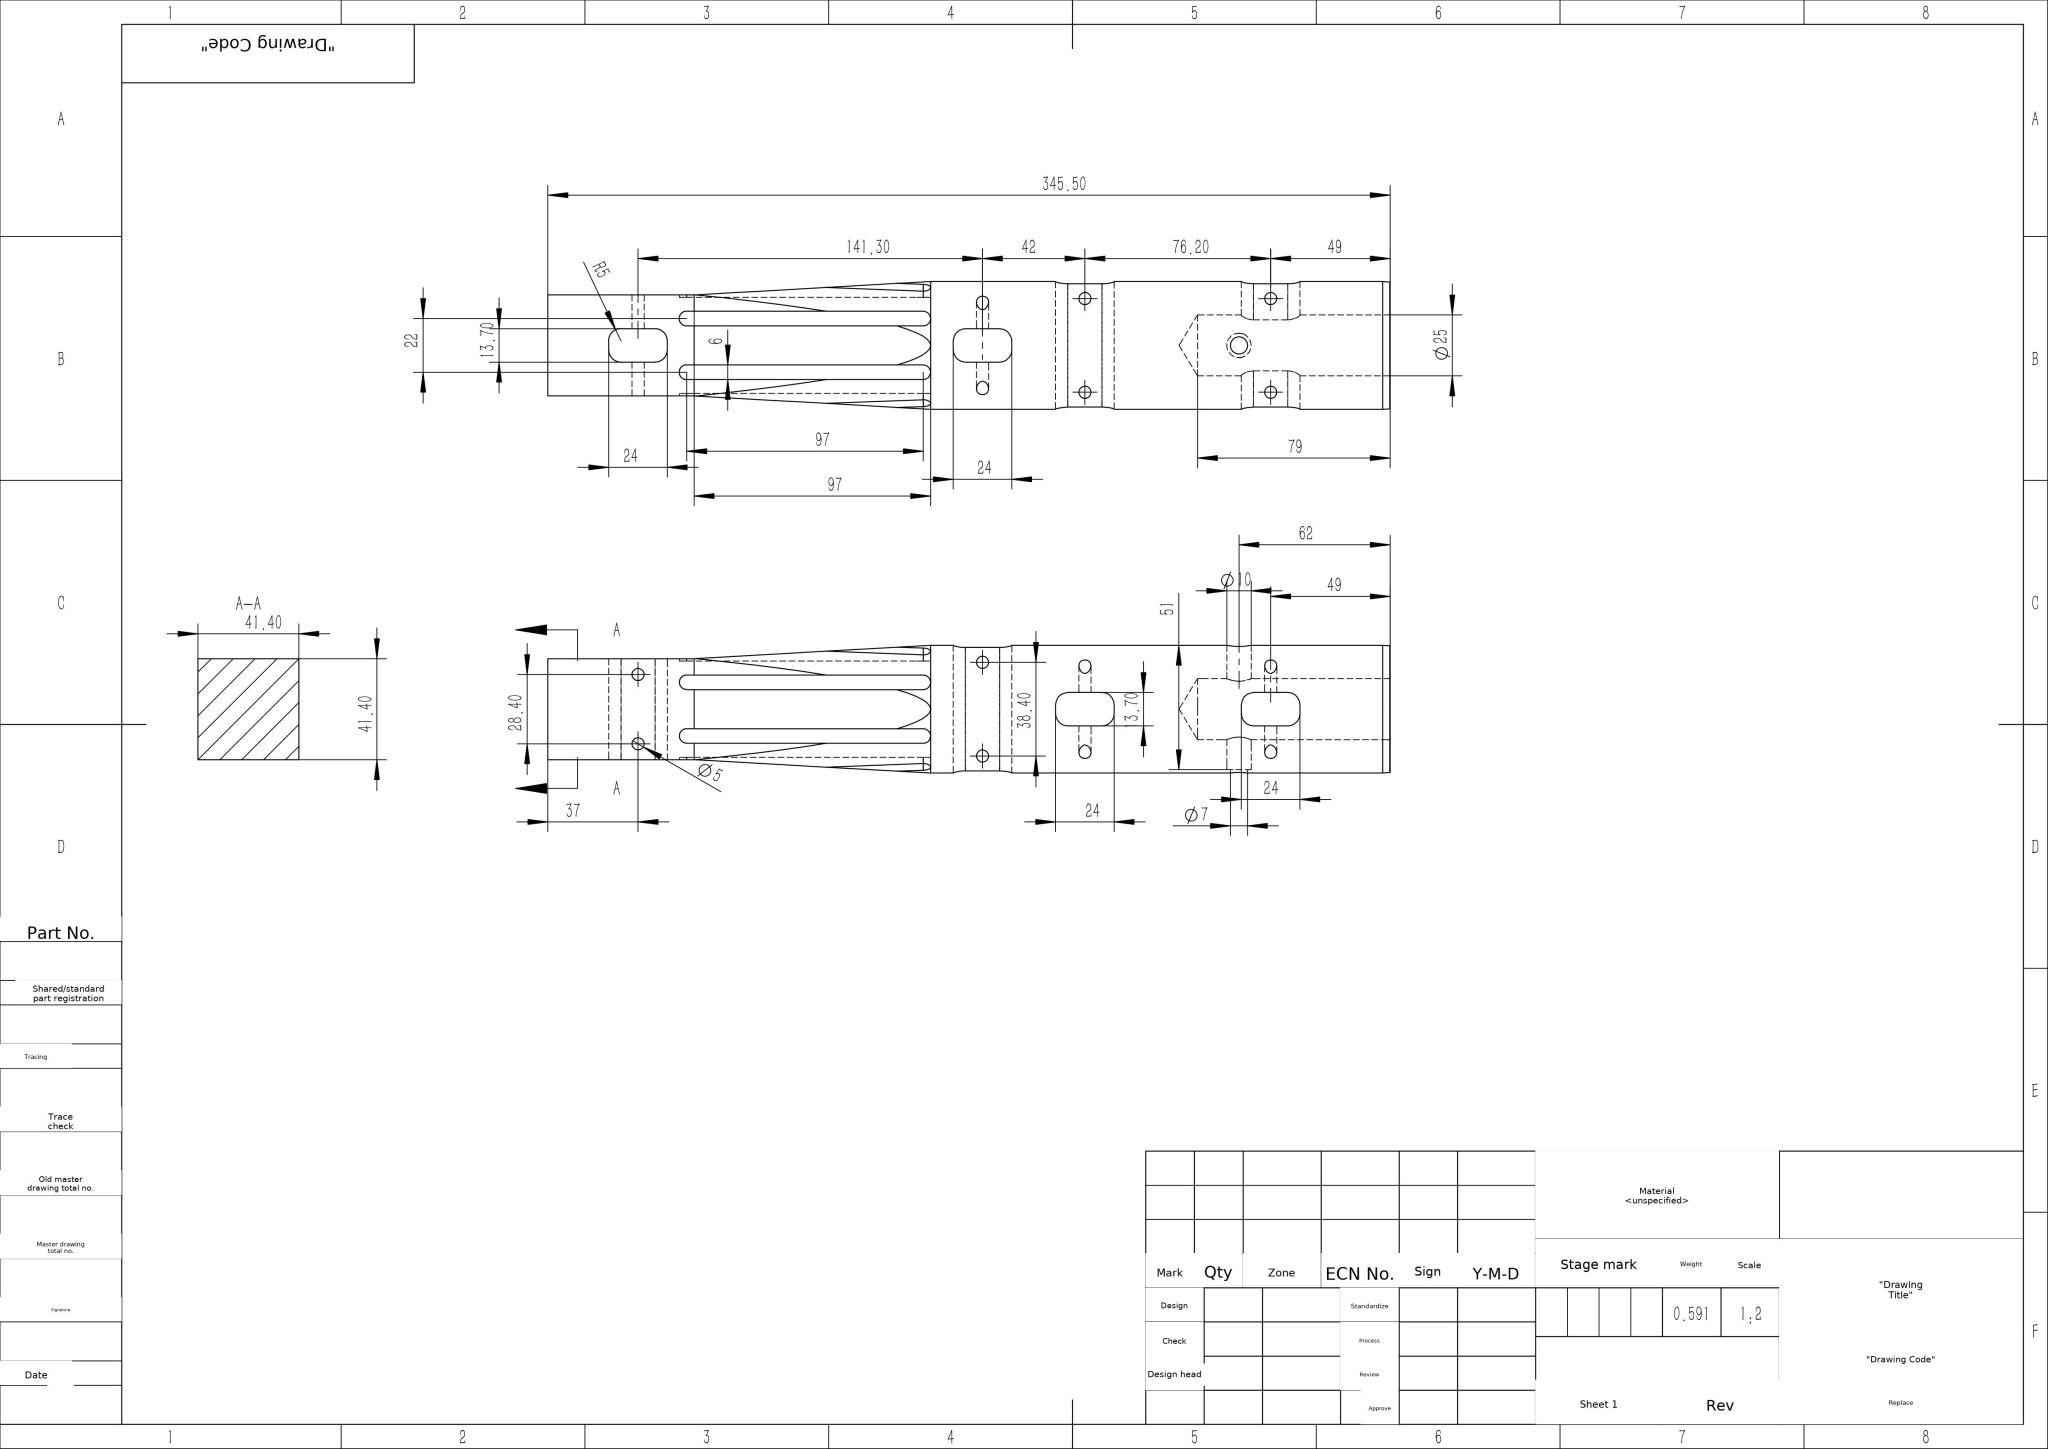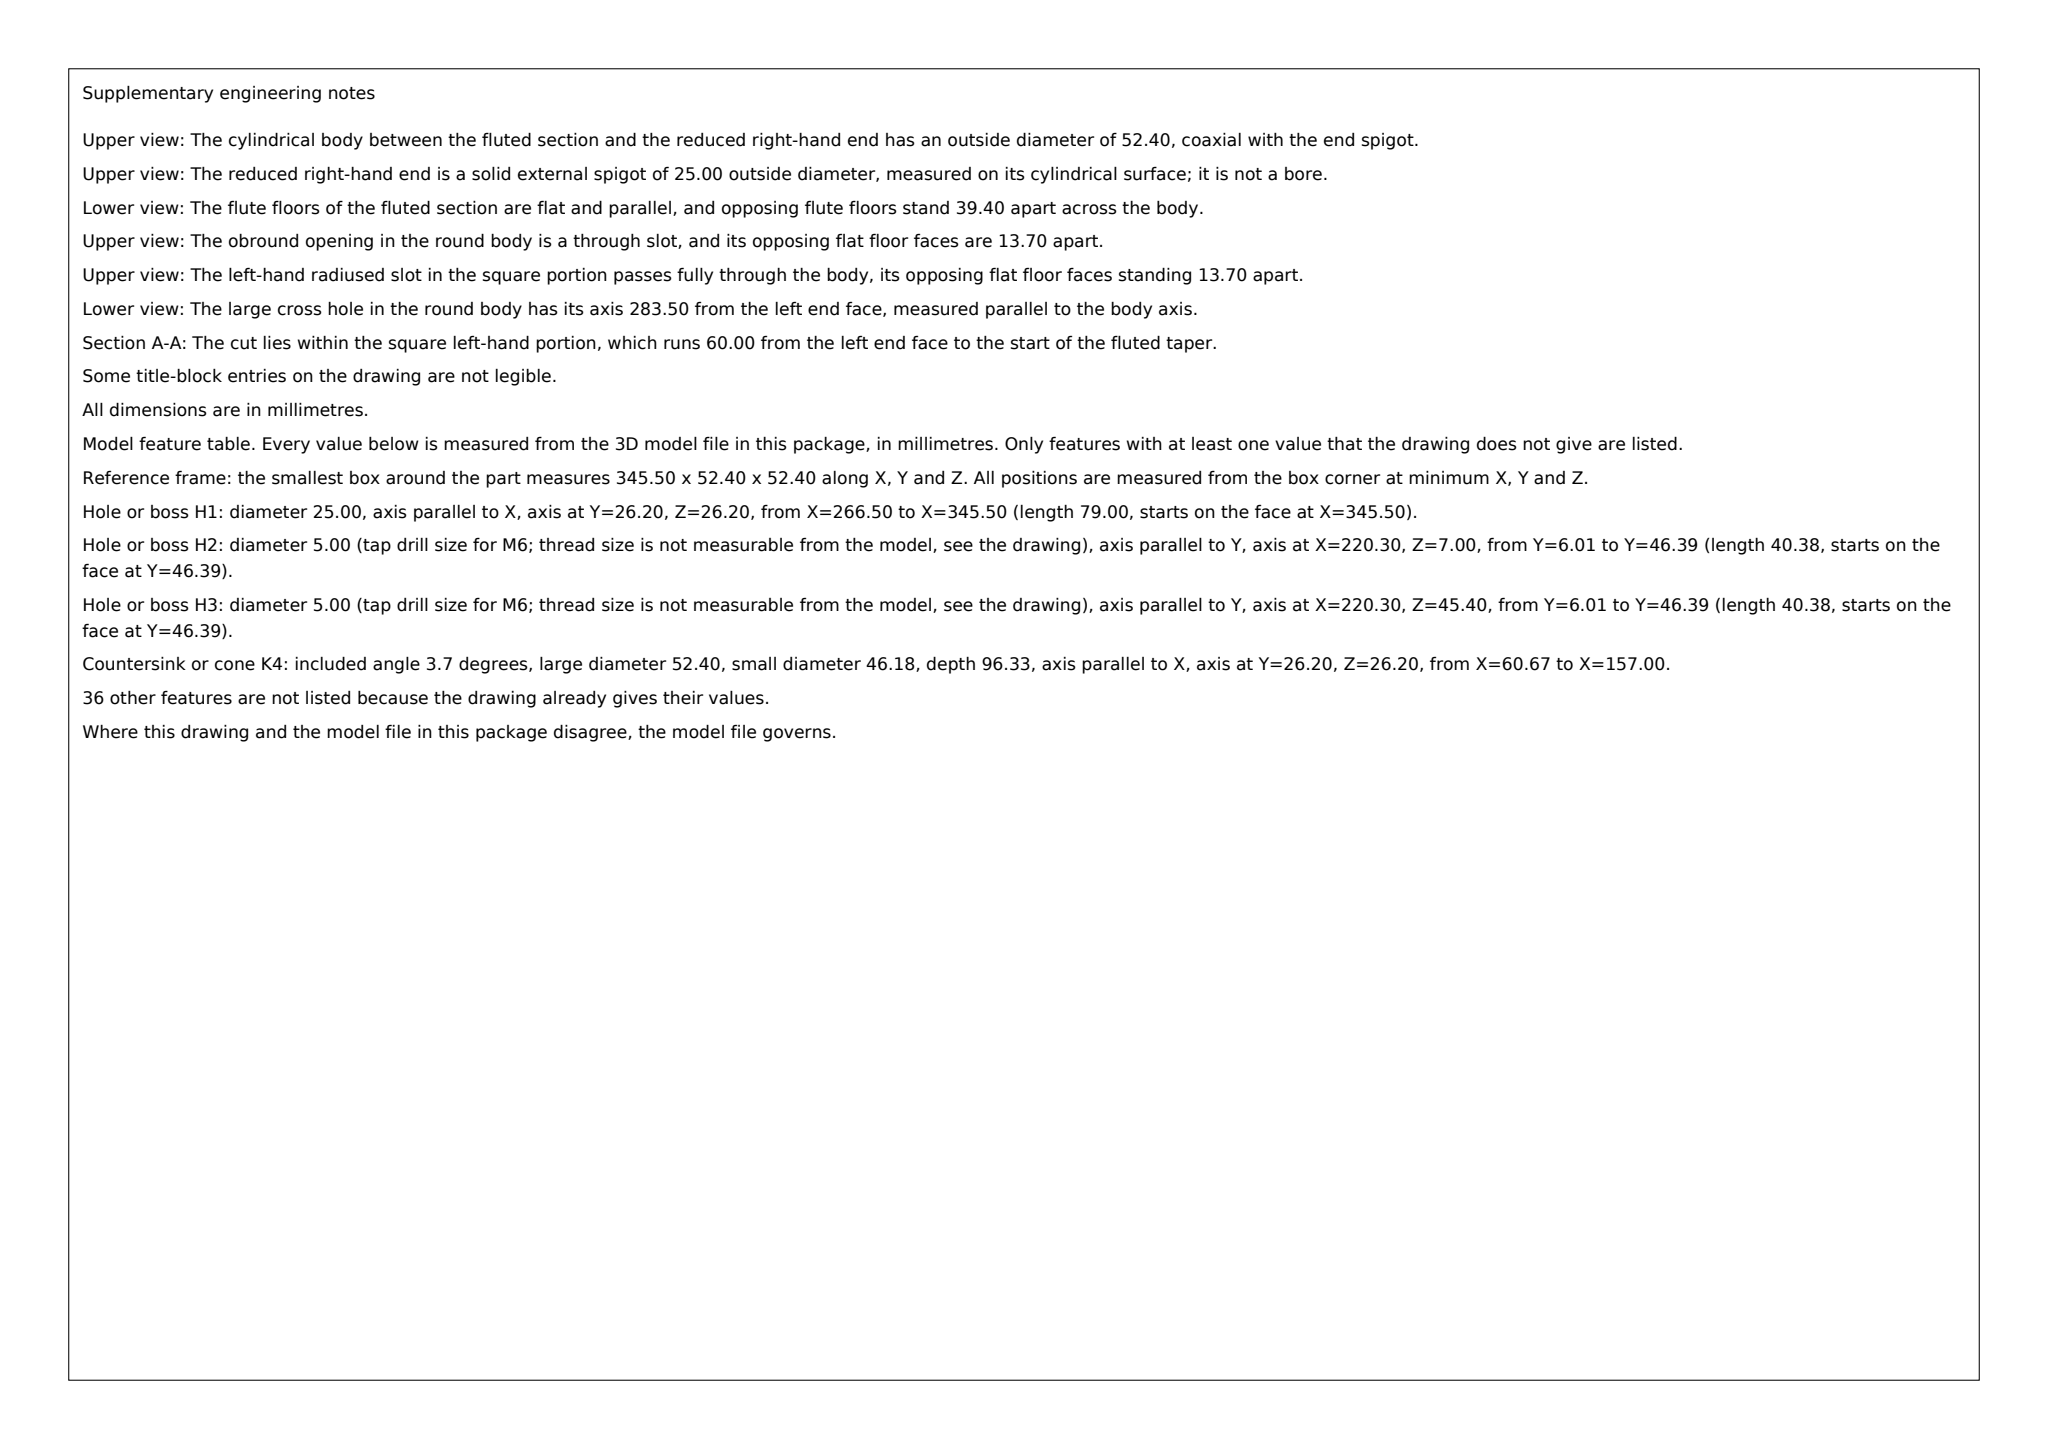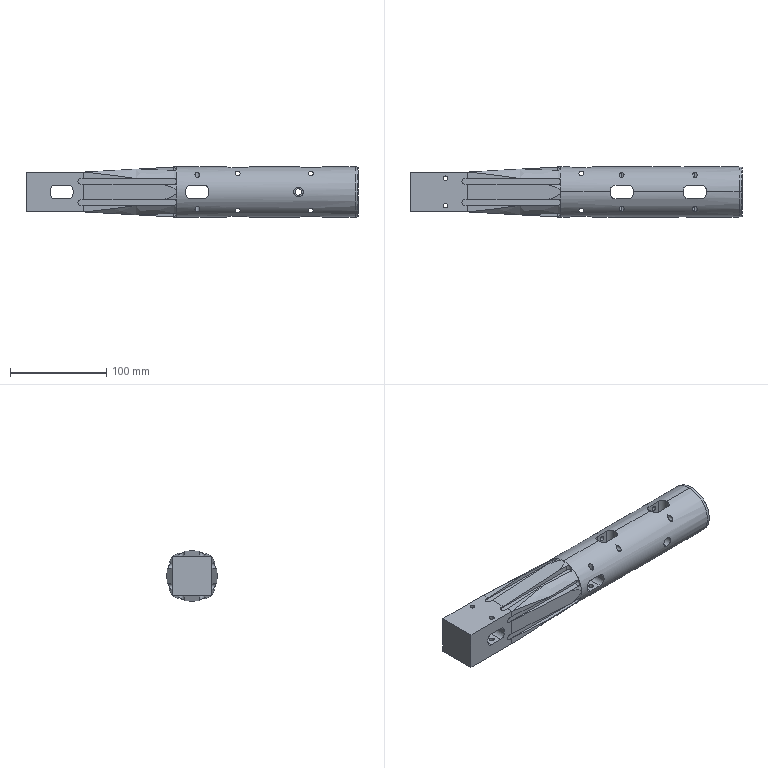Part | SolidWorks | mm | 1 solid | 159 faces | box 345.5 x 52.4 x 52.4 mm | volume 591419 mm3 | cylinder 78 | plane 63 | cone 16 | torus 2 | commonest cylinder face diameters 5 x32 10 x24 6 x16 7 x2 25 x2 52.4 x2
Drawing notes:
Ø52.40 SECTION TAPER: 8° INCL | from the solid: cones: [8.0, ref_dia 51.98, 2]
SLOT/FLANK RELIEF TAPERS: 3.7° INCL, 12 PL | from the solid: cones: [3.7, ref_dia 58.7, 12]
Ø25 BORE: 118° INCL POINT ANGLE | from the solid: cones: [118.0, ref_dia 25.0, 2]; Ø25 x-axis bore L=79
Ø6 RECESS DP 1.0 (8 PL) @ 57; DP 5.35 (8 PL) @ 154 FROM LH END | from the solid: cyl Ø6 len 1.0 at x=57 (y&z, 8 pl); Ø6 len 5.35 at x=154 (y&z, 8 pl)
UNSPECIFIED FILLETS R0.2 | from the solid: fillet_radii: [0.2, 2]
Ø5 DP 13.85 @ 37; Ø5 DP 13.34 ELSEWHERE, NOT THRU; Ø7 DP 1.4 | from the solid: Ø5 z-holes at x=37 len 13.85; other Ø5 len 13.34; Ø7 at x=283.5 len 1.4
Ø10 DP 13.34 FULL DIA (14.74 TO PT) BOTH SIDES, 62 FROM RH END | from the solid: Ø10 y-axis holes at x=283.5 (345.5-283.5=62), len 13.34 & 14.74, 2 ea side; Ø7 len 1.4 same axis
OVAL POCKET 24 x 13.70 DP 15.68, 2 PL BOTH FACES, 49 FROM RH END | from the solid: Ø10 z-axis cyls at x=289.5/303.5 (ctr 296.5 = 49 from 345.5), z ctrs 26.3/30.0, len 15.68, count 2 ea
Ø6 RECESS 8 PL (2 EA OF 4 FACES): 11 EA SIDE OF CL, 22 APART | from the solid: Ø6 holes at y/z = 17.15 & 39.15 vs section CL 28.15 → ±11.0; 4 at x=57 ↧1.0, 4 at x=154 ↧5.35
Ø52.40 ROUND SECTION: 185.50 LONG, EXTENDING FROM 160.00 FROM LH END TO RH END (345.50); SQUARE-TO-ROUND TRANSITION AT 160.00 FROM LH END | from the solid: cylinders: [52.4, axis x, length 185.5] combined with bbox_xyz x-length 345.5 (round section runs to RH end: 345.5 - 185.5 = 160.0)